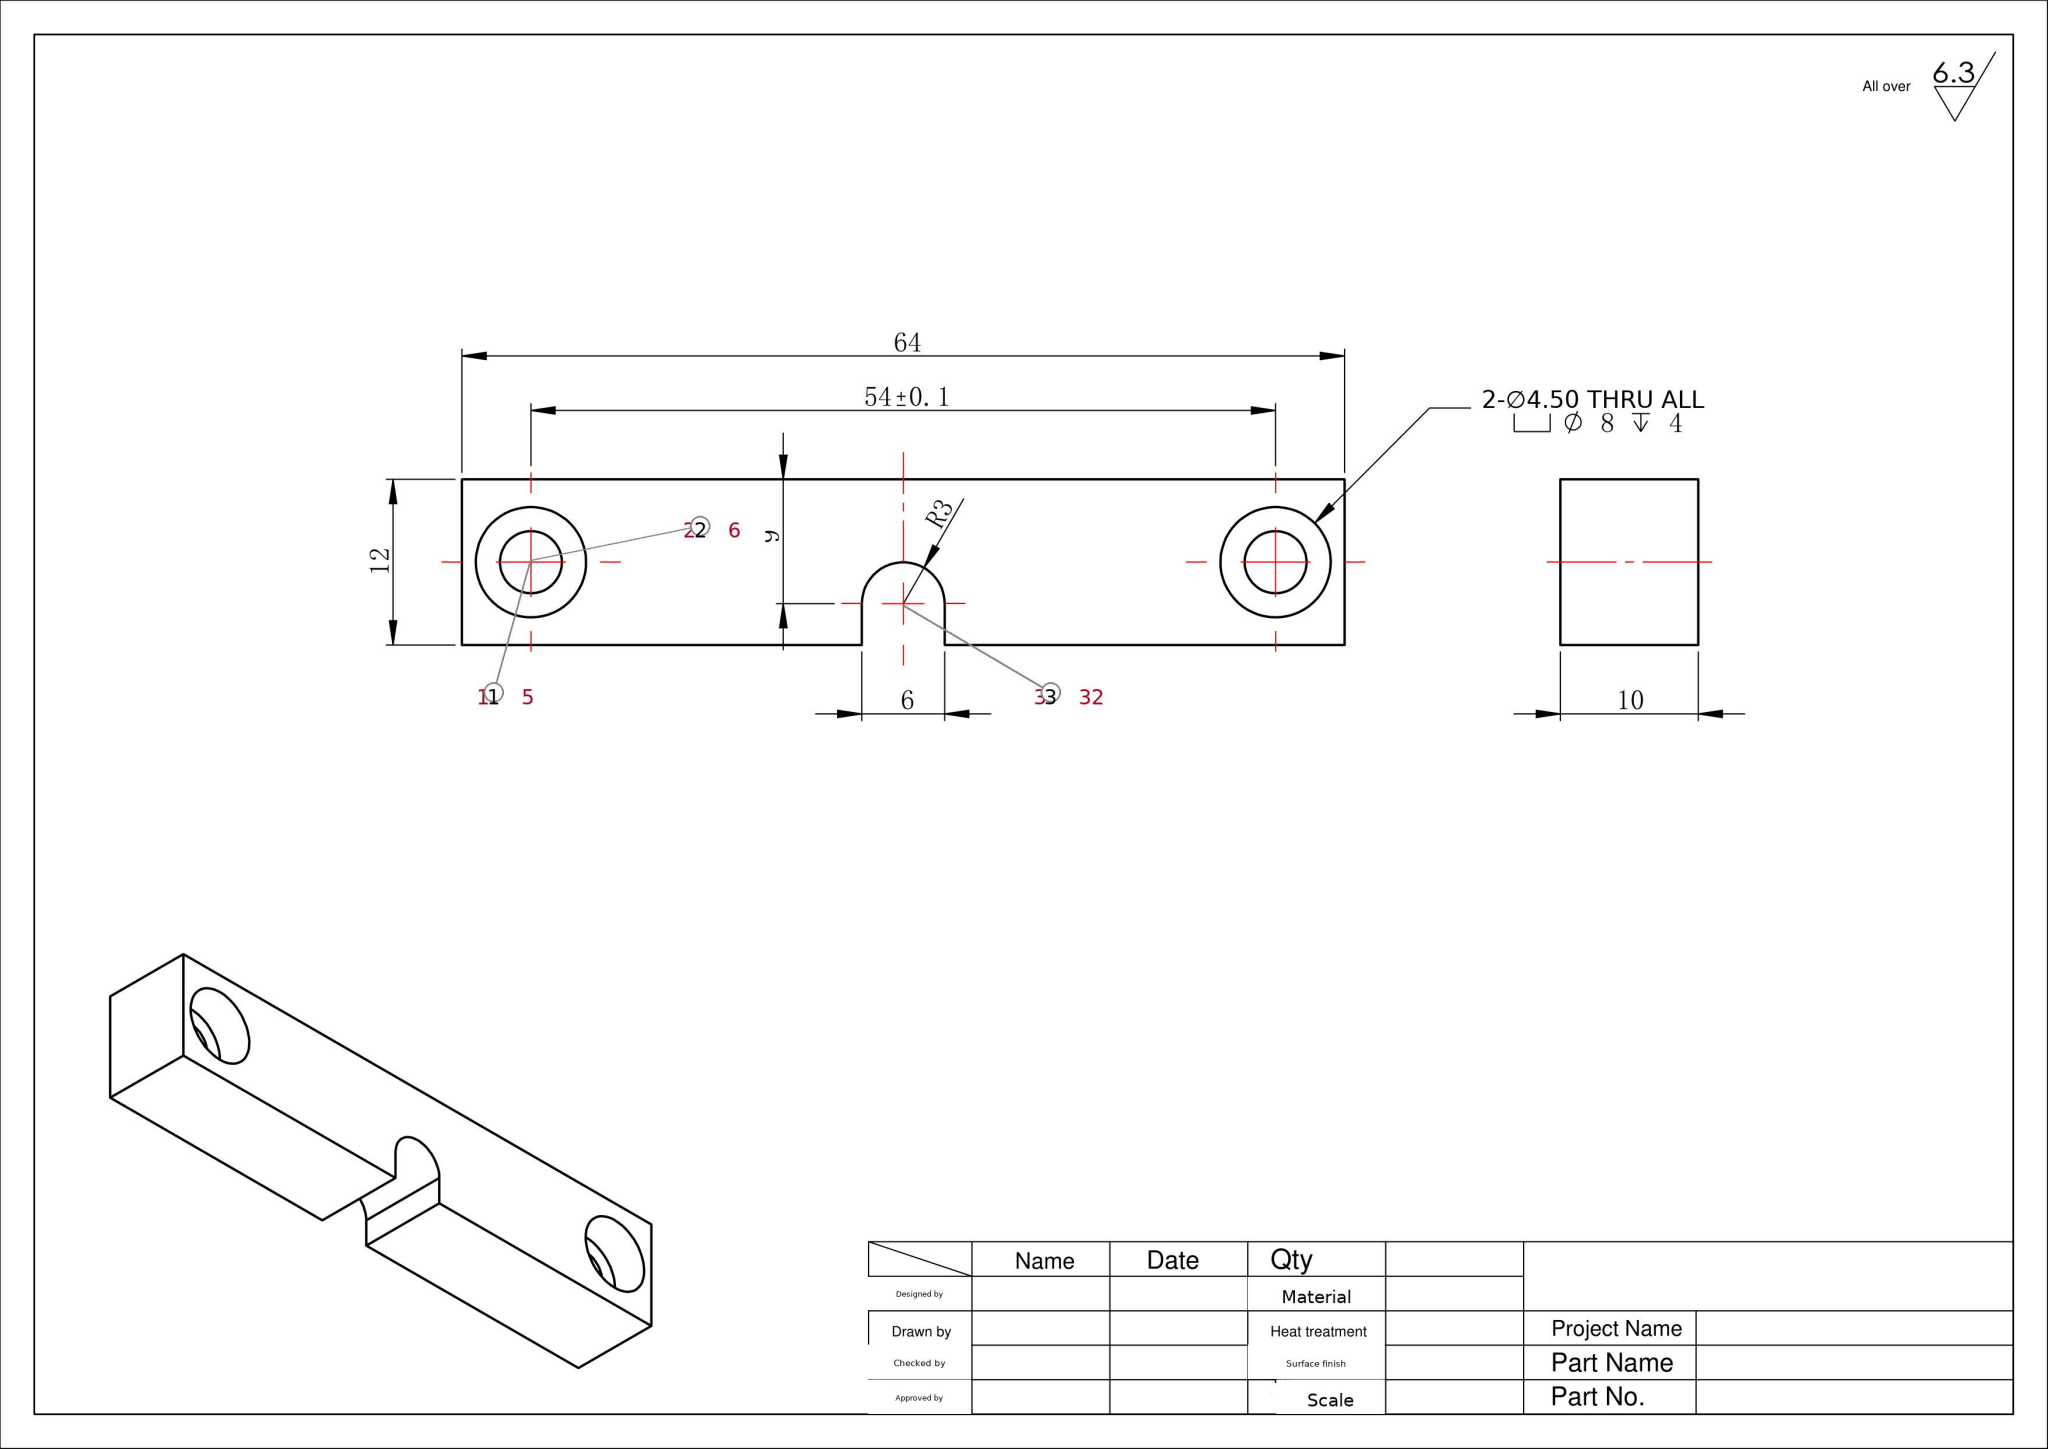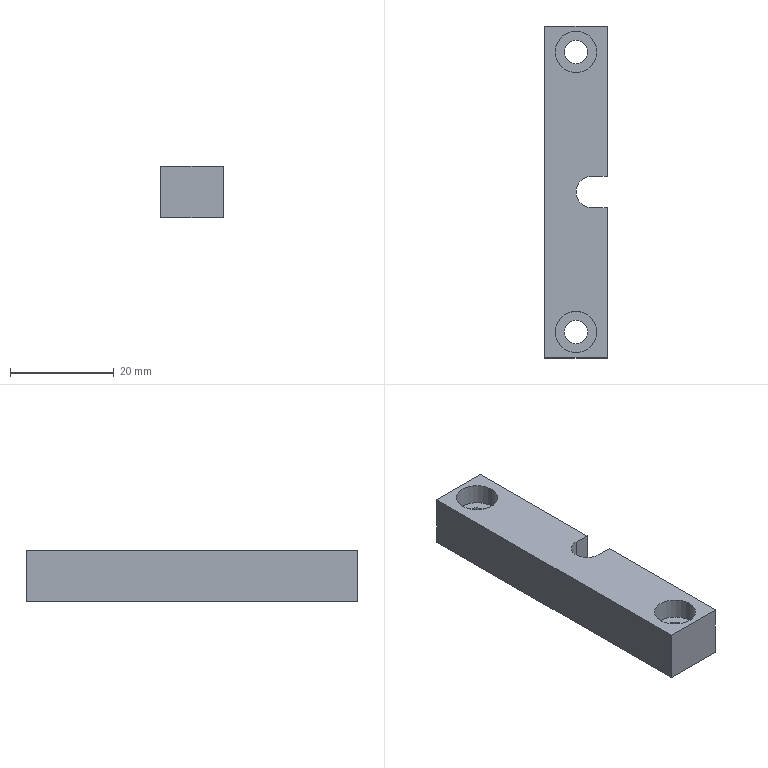Part | SolidWorks | mm | 1 solid | 20 faces | box 12 x 64 x 10 mm | volume 6766 mm3 | plane 11 | cylinder 9 | commonest cylinder face diameters 4.5 x4 8 x4 6 x1
build123d program:
from build123d import *

# Parameters (mm, degrees)
SKETCH1_W                                        = 12
SKETCH1_H                                        = 64
EXTRUDE1_DEPTH                                   = 10
CUT_EXTRUDE1_DEPTH                               = 66.879
M4_HEX_SOCKET_HEAD_CAP_SCREW_CBORE13_D           = 4.5
M4_HEX_SOCKET_HEAD_CAP_SCREW_CBORE13_CBORE_D     = 8
M4_HEX_SOCKET_HEAD_CAP_SCREW_CBORE13_CBORE_DEPTH = 4


with BuildPart() as part:
    # Sketch1 → Extrude1 (new body)
    with BuildSketch(Plane.XY):
        with Locations((6, 32)):
            Rectangle(SKETCH1_W, SKETCH1_H)
    extrude(amount=EXTRUDE1_DEPTH)

    # Sketch2 → Cut-Extrude1 (cut, through all)
    with BuildSketch(Plane.XY.offset(10)):
        with BuildLine():
            Line((9, 35), (14.637, 35))
            Line((14.637, 35), (14.637, 29))
            Line((14.637, 29), (9, 29))
            ThreePointArc((9, 29), (6, 32), (9, 35))
        make_face()
    extrude(amount=-CUT_EXTRUDE1_DEPTH, mode=Mode.SUBTRACT)

    # M4 Hex Socket Head Cap Screw CBORE13 (through all)
    with Locations(Plane(origin=(6, 59, 10), x_dir=(1, 0, 0), z_dir=(0, 0, 1))):
        with Locations((0, 0), (0, -54)):
            CounterBoreHole(M4_HEX_SOCKET_HEAD_CAP_SCREW_CBORE13_D / 2, M4_HEX_SOCKET_HEAD_CAP_SCREW_CBORE13_CBORE_D / 2, M4_HEX_SOCKET_HEAD_CAP_SCREW_CBORE13_CBORE_DEPTH)


solid = part.part
STEP:
#1=CARTESIAN_POINT('',(3.75,59.,0.));
#2=VERTEX_POINT('',#1);
#3=CARTESIAN_POINT('',(8.25,59.,0.));
#4=VERTEX_POINT('',#3);
#5=CARTESIAN_POINT('',(6.,59.,0.));
#6=DIRECTION('',(0.,0.,1.));
#7=DIRECTION('',(1.,0.,0.));
#8=AXIS2_PLACEMENT_3D('',#5,#6,#7);
#9=CIRCLE('',#8,2.25);
#10=EDGE_CURVE('',#2,#4,#9,.T.);
#11=ORIENTED_EDGE('',*,*,#10,.F.);
#12=CARTESIAN_POINT('',(3.75,59.,6.));
#13=VERTEX_POINT('',#12);
#14=CARTESIAN_POINT('',(3.75,59.,10.));
#15=DIRECTION('',(0.,0.,1.));
#16=VECTOR('',#15,1000.);
#17=LINE('',#14,#16);
#18=EDGE_CURVE('',#2,#13,#17,.T.);
#19=ORIENTED_EDGE('',*,*,#18,.T.);
#20=CARTESIAN_POINT('',(8.25,59.,6.));
#21=VERTEX_POINT('',#20);
#22=CARTESIAN_POINT('',(6.,59.,6.));
#23=DIRECTION('',(0.,0.,1.));
#24=DIRECTION('',(1.,0.,0.));
#25=AXIS2_PLACEMENT_3D('',#22,#23,#24);
#26=CIRCLE('',#25,2.25);
#27=EDGE_CURVE('',#13,#21,#26,.T.);
#28=ORIENTED_EDGE('',*,*,#27,.T.);
#29=CARTESIAN_POINT('',(8.25,59.,10.));
#30=DIRECTION('',(0.,0.,1.));
#31=VECTOR('',#30,1000.);
#32=LINE('',#29,#31);
#33=EDGE_CURVE('',#4,#21,#32,.T.);
#34=ORIENTED_EDGE('',*,*,#33,.F.);
#35=EDGE_LOOP('',(#11,#19,#28,#34));
#36=FACE_OUTER_BOUND('',#35,.T.);
#37=CARTESIAN_POINT('',(6.,59.,10.));
#38=DIRECTION('',(0.,0.,1.));
#39=DIRECTION('',(1.,0.,0.));
#40=AXIS2_PLACEMENT_3D('',#37,#38,#39);
#41=CYLINDRICAL_SURFACE('',#40,2.25);
#42=ADVANCED_FACE('',(#36),#41,.F.);
#43=CARTESIAN_POINT('',(2.,59.,6.));
#44=VERTEX_POINT('',#43);
#45=CARTESIAN_POINT('',(10.,59.,6.));
#46=VERTEX_POINT('',#45);
#47=CARTESIAN_POINT('',(6.,59.,6.));
#48=DIRECTION('',(0.,0.,1.));
#49=DIRECTION('',(1.,0.,0.));
#50=AXIS2_PLACEMENT_3D('',#47,#48,#49);
#51=CIRCLE('',#50,4.);
#52=EDGE_CURVE('',#44,#46,#51,.T.);
#53=ORIENTED_EDGE('',*,*,#52,.F.);
#54=CARTESIAN_POINT('',(2.,59.,10.));
#55=VERTEX_POINT('',#54);
#56=CARTESIAN_POINT('',(2.,59.,10.));
#57=DIRECTION('',(0.,0.,1.));
#58=VECTOR('',#57,1000.);
#59=LINE('',#56,#58);
#60=EDGE_CURVE('',#44,#55,#59,.T.);
#61=ORIENTED_EDGE('',*,*,#60,.T.);
#62=CARTESIAN_POINT('',(10.,59.,10.));
#63=VERTEX_POINT('',#62);
#64=CARTESIAN_POINT('',(6.,59.,10.));
#65=DIRECTION('',(0.,0.,1.));
#66=DIRECTION('',(1.,0.,0.));
#67=AXIS2_PLACEMENT_3D('',#64,#65,#66);
#68=CIRCLE('',#67,4.);
#69=EDGE_CURVE('',#55,#63,#68,.T.);
#70=ORIENTED_EDGE('',*,*,#69,.T.);
#71=CARTESIAN_POINT('',(10.,59.,10.));
#72=DIRECTION('',(0.,0.,1.));
#73=VECTOR('',#72,1000.);
#74=LINE('',#71,#73);
#75=EDGE_CURVE('',#46,#63,#74,.T.);
#76=ORIENTED_EDGE('',*,*,#75,.F.);
#77=EDGE_LOOP('',(#53,#61,#70,#76));
#78=FACE_OUTER_BOUND('',#77,.T.);
#79=CARTESIAN_POINT('',(6.,59.,10.));
#80=DIRECTION('',(0.,0.,1.));
#81=DIRECTION('',(1.,0.,0.));
#82=AXIS2_PLACEMENT_3D('',#79,#80,#81);
#83=CYLINDRICAL_SURFACE('',#82,4.);
#84=ADVANCED_FACE('',(#78),#83,.F.);
#85=CARTESIAN_POINT('',(3.75,5.,0.));
#86=VERTEX_POINT('',#85);
#87=CARTESIAN_POINT('',(8.25,5.,0.));
#88=VERTEX_POINT('',#87);
#89=CARTESIAN_POINT('',(6.,5.,0.));
#90=DIRECTION('',(0.,0.,1.));
#91=DIRECTION('',(1.,0.,0.));
#92=AXIS2_PLACEMENT_3D('',#89,#90,#91);
#93=CIRCLE('',#92,2.25);
#94=EDGE_CURVE('',#86,#88,#93,.T.);
#95=ORIENTED_EDGE('',*,*,#94,.F.);
#96=CARTESIAN_POINT('',(3.75,5.,6.));
#97=VERTEX_POINT('',#96);
#98=CARTESIAN_POINT('',(3.75,5.,10.));
#99=DIRECTION('',(0.,0.,1.));
#100=VECTOR('',#99,1000.);
#101=LINE('',#98,#100);
#102=EDGE_CURVE('',#86,#97,#101,.T.);
#103=ORIENTED_EDGE('',*,*,#102,.T.);
#104=CARTESIAN_POINT('',(8.25,5.,6.));
#105=VERTEX_POINT('',#104);
#106=CARTESIAN_POINT('',(6.,5.,6.));
#107=DIRECTION('',(0.,0.,1.));
#108=DIRECTION('',(1.,0.,0.));
#109=AXIS2_PLACEMENT_3D('',#106,#107,#108);
#110=CIRCLE('',#109,2.25);
#111=EDGE_CURVE('',#97,#105,#110,.T.);
#112=ORIENTED_EDGE('',*,*,#111,.T.);
#113=CARTESIAN_POINT('',(8.25,5.,10.));
#114=DIRECTION('',(0.,0.,1.));
#115=VECTOR('',#114,1000.);
#116=LINE('',#113,#115);
#117=EDGE_CURVE('',#88,#105,#116,.T.);
#118=ORIENTED_EDGE('',*,*,#117,.F.);
#119=EDGE_LOOP('',(#95,#103,#112,#118));
#120=FACE_OUTER_BOUND('',#119,.T.);
#121=CARTESIAN_POINT('',(6.,5.,10.));
#122=DIRECTION('',(0.,0.,1.));
#123=DIRECTION('',(1.,0.,0.));
#124=AXIS2_PLACEMENT_3D('',#121,#122,#123);
#125=CYLINDRICAL_SURFACE('',#124,2.25);
#126=ADVANCED_FACE('',(#120),#125,.F.);
#127=CARTESIAN_POINT('',(2.,5.,6.));
#128=VERTEX_POINT('',#127);
#129=CARTESIAN_POINT('',(10.,5.,6.));
#130=VERTEX_POINT('',#129);
#131=CARTESIAN_POINT('',(6.,5.,6.));
#132=DIRECTION('',(0.,0.,1.));
#133=DIRECTION('',(1.,0.,0.));
#134=AXIS2_PLACEMENT_3D('',#131,#132,#133);
#135=CIRCLE('',#134,4.);
#136=EDGE_CURVE('',#128,#130,#135,.T.);
#137=ORIENTED_EDGE('',*,*,#136,.F.);
#138=CARTESIAN_POINT('',(2.,5.,10.));
#139=VERTEX_POINT('',#138);
#140=CARTESIAN_POINT('',(2.,5.,10.));
#141=DIRECTION('',(0.,0.,1.));
#142=VECTOR('',#141,1000.);
#143=LINE('',#140,#142);
#144=EDGE_CURVE('',#128,#139,#143,.T.);
#145=ORIENTED_EDGE('',*,*,#144,.T.);
#146=CARTESIAN_POINT('',(10.,5.,10.));
#147=VERTEX_POINT('',#146);
#148=CARTESIAN_POINT('',(6.,5.,10.));
#149=DIRECTION('',(0.,0.,1.));
#150=DIRECTION('',(1.,0.,0.));
#151=AXIS2_PLACEMENT_3D('',#148,#149,#150);
#152=CIRCLE('',#151,4.);
#153=EDGE_CURVE('',#139,#147,#152,.T.);
#154=ORIENTED_EDGE('',*,*,#153,.T.);
#155=CARTESIAN_POINT('',(10.,5.,10.));
#156=DIRECTION('',(0.,0.,1.));
#157=VECTOR('',#156,1000.);
#158=LINE('',#155,#157);
#159=EDGE_CURVE('',#130,#147,#158,.T.);
#160=ORIENTED_EDGE('',*,*,#159,.F.);
#161=EDGE_LOOP('',(#137,#145,#154,#160));
#162=FACE_OUTER_BOUND('',#161,.T.);
#163=CARTESIAN_POINT('',(6.,5.,10.));
#164=DIRECTION('',(0.,0.,1.));
#165=DIRECTION('',(1.,0.,0.));
#166=AXIS2_PLACEMENT_3D('',#163,#164,#165);
#167=CYLINDRICAL_SURFACE('',#166,4.);
#168=ADVANCED_FACE('',(#162),#167,.F.);
#169=CARTESIAN_POINT('',(12.,35.,10.));
#170=VERTEX_POINT('',#169);
#171=CARTESIAN_POINT('',(12.,64.,10.));
#172=VERTEX_POINT('',#171);
#173=CARTESIAN_POINT('',(12.,0.,10.));
#174=DIRECTION('',(0.,1.,0.));
#175=VECTOR('',#174,1000.);
#176=LINE('',#173,#175);
#177=EDGE_CURVE('',#170,#172,#176,.T.);
#178=ORIENTED_EDGE('',*,*,#177,.F.);
#179=CARTESIAN_POINT('',(12.,35.,0.));
#180=VERTEX_POINT('',#179);
#181=CARTESIAN_POINT('',(12.,35.,10.));
#182=DIRECTION('',(0.,0.,-1.));
#183=VECTOR('',#182,1000.);
#184=LINE('',#181,#183);
#185=EDGE_CURVE('',#170,#180,#184,.T.);
#186=ORIENTED_EDGE('',*,*,#185,.T.);
#187=CARTESIAN_POINT('',(12.,64.,0.));
#188=VERTEX_POINT('',#187);
#189=CARTESIAN_POINT('',(12.,0.,0.));
#190=DIRECTION('',(0.,1.,0.));
#191=VECTOR('',#190,1000.);
#192=LINE('',#189,#191);
#193=EDGE_CURVE('',#180,#188,#192,.T.);
#194=ORIENTED_EDGE('',*,*,#193,.T.);
#195=CARTESIAN_POINT('',(12.,64.,10.));
#196=DIRECTION('',(0.,0.,-1.));
#197=VECTOR('',#196,1000.);
#198=LINE('',#195,#197);
#199=EDGE_CURVE('',#172,#188,#198,.T.);
#200=ORIENTED_EDGE('',*,*,#199,.F.);
#201=EDGE_LOOP('',(#178,#186,#194,#200));
#202=FACE_OUTER_BOUND('',#201,.T.);
#203=CARTESIAN_POINT('',(12.,0.,10.));
#204=DIRECTION('',(-1.,0.,0.));
#205=DIRECTION('',(0.,0.,1.));
#206=AXIS2_PLACEMENT_3D('',#203,#204,#205);
#207=PLANE('',#206);
#208=ADVANCED_FACE('',(#202),#207,.F.);
#209=CARTESIAN_POINT('',(0.,64.,0.));
#210=VERTEX_POINT('',#209);
#211=CARTESIAN_POINT('',(0.,0.,0.));
#212=VERTEX_POINT('',#211);
#213=CARTESIAN_POINT('',(0.,0.,0.));
#214=DIRECTION('',(0.,-1.,0.));
#215=VECTOR('',#214,1000.);
#216=LINE('',#213,#215);
#217=EDGE_CURVE('',#210,#212,#216,.T.);
#218=ORIENTED_EDGE('',*,*,#217,.T.);
#219=CARTESIAN_POINT('',(0.,0.,10.));
#220=VERTEX_POINT('',#219);
#221=CARTESIAN_POINT('',(0.,0.,10.));
#222=DIRECTION('',(0.,0.,-1.));
#223=VECTOR('',#222,1000.);
#224=LINE('',#221,#223);
#225=EDGE_CURVE('',#220,#212,#224,.T.);
#226=ORIENTED_EDGE('',*,*,#225,.F.);
#227=CARTESIAN_POINT('',(0.,64.,10.));
#228=VERTEX_POINT('',#227);
#229=CARTESIAN_POINT('',(0.,0.,10.));
#230=DIRECTION('',(0.,-1.,0.));
#231=VECTOR('',#230,1000.);
#232=LINE('',#229,#231);
#233=EDGE_CURVE('',#228,#220,#232,.T.);
#234=ORIENTED_EDGE('',*,*,#233,.F.);
#235=CARTESIAN_POINT('',(0.,64.,10.));
#236=DIRECTION('',(0.,0.,-1.));
#237=VECTOR('',#236,1000.);
#238=LINE('',#235,#237);
#239=EDGE_CURVE('',#228,#210,#238,.T.);
#240=ORIENTED_EDGE('',*,*,#239,.T.);
#241=EDGE_LOOP('',(#218,#226,#234,#240));
#242=FACE_OUTER_BOUND('',#241,.T.);
#243=CARTESIAN_POINT('',(0.,0.,10.));
#244=DIRECTION('',(1.,0.,0.));
#245=DIRECTION('',(0.,0.,-1.));
#246=AXIS2_PLACEMENT_3D('',#243,#244,#245);
#247=PLANE('',#246);
#248=ADVANCED_FACE('',(#242),#247,.F.);
#249=CARTESIAN_POINT('',(12.,0.,0.));
#250=VERTEX_POINT('',#249);
#251=CARTESIAN_POINT('',(0.,0.,0.));
#252=DIRECTION('',(1.,0.,0.));
#253=VECTOR('',#252,1000.);
#254=LINE('',#251,#253);
#255=EDGE_CURVE('',#212,#250,#254,.T.);
#256=ORIENTED_EDGE('',*,*,#255,.T.);
#257=CARTESIAN_POINT('',(12.,0.,10.));
#258=VERTEX_POINT('',#257);
#259=CARTESIAN_POINT('',(12.,0.,10.));
#260=DIRECTION('',(0.,0.,-1.));
#261=VECTOR('',#260,1000.);
#262=LINE('',#259,#261);
#263=EDGE_CURVE('',#258,#250,#262,.T.);
#264=ORIENTED_EDGE('',*,*,#263,.F.);
#265=CARTESIAN_POINT('',(0.,0.,10.));
#266=DIRECTION('',(1.,0.,0.));
#267=VECTOR('',#266,1000.);
#268=LINE('',#265,#267);
#269=EDGE_CURVE('',#220,#258,#268,.T.);
#270=ORIENTED_EDGE('',*,*,#269,.F.);
#271=ORIENTED_EDGE('',*,*,#225,.T.);
#272=EDGE_LOOP('',(#256,#264,#270,#271));
#273=FACE_OUTER_BOUND('',#272,.T.);
#274=CARTESIAN_POINT('',(0.,0.,10.));
#275=DIRECTION('',(0.,1.,0.));
#276=DIRECTION('',(0.,0.,1.));
#277=AXIS2_PLACEMENT_3D('',#274,#275,#276);
#278=PLANE('',#277);
#279=ADVANCED_FACE('',(#273),#278,.F.);
#280=CARTESIAN_POINT('',(12.,29.,0.));
#281=VERTEX_POINT('',#280);
#282=CARTESIAN_POINT('',(12.,0.,0.));
#283=DIRECTION('',(0.,1.,0.));
#284=VECTOR('',#283,1000.);
#285=LINE('',#282,#284);
#286=EDGE_CURVE('',#250,#281,#285,.T.);
#287=ORIENTED_EDGE('',*,*,#286,.T.);
#288=CARTESIAN_POINT('',(12.,29.,10.));
#289=VERTEX_POINT('',#288);
#290=CARTESIAN_POINT('',(12.,29.,10.));
#291=DIRECTION('',(0.,0.,1.));
#292=VECTOR('',#291,1000.);
#293=LINE('',#290,#292);
#294=EDGE_CURVE('',#281,#289,#293,.T.);
#295=ORIENTED_EDGE('',*,*,#294,.T.);
#296=CARTESIAN_POINT('',(12.,0.,10.));
#297=DIRECTION('',(0.,1.,0.));
#298=VECTOR('',#297,1000.);
#299=LINE('',#296,#298);
#300=EDGE_CURVE('',#258,#289,#299,.T.);
#301=ORIENTED_EDGE('',*,*,#300,.F.);
#302=ORIENTED_EDGE('',*,*,#263,.T.);
#303=EDGE_LOOP('',(#287,#295,#301,#302));
#304=FACE_OUTER_BOUND('',#303,.T.);
#305=CARTESIAN_POINT('',(12.,0.,10.));
#306=DIRECTION('',(-1.,0.,0.));
#307=DIRECTION('',(0.,0.,1.));
#308=AXIS2_PLACEMENT_3D('',#305,#306,#307);
#309=PLANE('',#308);
#310=ADVANCED_FACE('',(#304),#309,.F.);
#311=CARTESIAN_POINT('',(0.,64.,0.));
#312=DIRECTION('',(-1.,0.,0.));
#313=VECTOR('',#312,1000.);
#314=LINE('',#311,#313);
#315=EDGE_CURVE('',#188,#210,#314,.T.);
#316=ORIENTED_EDGE('',*,*,#315,.T.);
#317=ORIENTED_EDGE('',*,*,#239,.F.);
#318=CARTESIAN_POINT('',(0.,64.,10.));
#319=DIRECTION('',(-1.,0.,0.));
#320=VECTOR('',#319,1000.);
#321=LINE('',#318,#320);
#322=EDGE_CURVE('',#172,#228,#321,.T.);
#323=ORIENTED_EDGE('',*,*,#322,.F.);
#324=ORIENTED_EDGE('',*,*,#199,.T.);
#325=EDGE_LOOP('',(#316,#317,#323,#324));
#326=FACE_OUTER_BOUND('',#325,.T.);
#327=CARTESIAN_POINT('',(0.,64.,10.));
#328=DIRECTION('',(0.,-1.,0.));
#329=DIRECTION('',(0.,0.,-1.));
#330=AXIS2_PLACEMENT_3D('',#327,#328,#329);
#331=PLANE('',#330);
#332=ADVANCED_FACE('',(#326),#331,.F.);
#333=CARTESIAN_POINT('',(6.,59.,10.));
#334=DIRECTION('',(0.,0.,1.));
#335=DIRECTION('',(1.,0.,0.));
#336=AXIS2_PLACEMENT_3D('',#333,#334,#335);
#337=CIRCLE('',#336,4.);
#338=EDGE_CURVE('',#63,#55,#337,.T.);
#339=ORIENTED_EDGE('',*,*,#338,.F.);
#340=ORIENTED_EDGE('',*,*,#69,.F.);
#341=EDGE_LOOP('',(#339,#340));
#342=FACE_BOUND('',#341,.T.);
#343=CARTESIAN_POINT('',(6.,5.,10.));
#344=DIRECTION('',(0.,0.,1.));
#345=DIRECTION('',(1.,0.,0.));
#346=AXIS2_PLACEMENT_3D('',#343,#344,#345);
#347=CIRCLE('',#346,4.);
#348=EDGE_CURVE('',#147,#139,#347,.T.);
#349=ORIENTED_EDGE('',*,*,#348,.F.);
#350=ORIENTED_EDGE('',*,*,#153,.F.);
#351=EDGE_LOOP('',(#349,#350));
#352=FACE_BOUND('',#351,.T.);
#353=CARTESIAN_POINT('',(9.,35.,10.));
#354=VERTEX_POINT('',#353);
#355=CARTESIAN_POINT('',(9.,29.,10.));
#356=VERTEX_POINT('',#355);
#357=CARTESIAN_POINT('',(9.,32.,10.));
#358=DIRECTION('',(0.,0.,1.));
#359=DIRECTION('',(1.,0.,0.));
#360=AXIS2_PLACEMENT_3D('',#357,#358,#359);
#361=CIRCLE('',#360,3.);
#362=EDGE_CURVE('',#354,#356,#361,.T.);
#363=ORIENTED_EDGE('',*,*,#362,.F.);
#364=CARTESIAN_POINT('',(9.,35.,10.));
#365=DIRECTION('',(-1.,0.,0.));
#366=VECTOR('',#365,1000.);
#367=LINE('',#364,#366);
#368=EDGE_CURVE('',#170,#354,#367,.T.);
#369=ORIENTED_EDGE('',*,*,#368,.F.);
#370=ORIENTED_EDGE('',*,*,#177,.T.);
#371=ORIENTED_EDGE('',*,*,#322,.T.);
#372=ORIENTED_EDGE('',*,*,#233,.T.);
#373=ORIENTED_EDGE('',*,*,#269,.T.);
#374=ORIENTED_EDGE('',*,*,#300,.T.);
#375=CARTESIAN_POINT('',(14.637,29.,10.));
#376=DIRECTION('',(1.,0.,0.));
#377=VECTOR('',#376,1000.);
#378=LINE('',#375,#377);
#379=EDGE_CURVE('',#356,#289,#378,.T.);
#380=ORIENTED_EDGE('',*,*,#379,.F.);
#381=EDGE_LOOP('',(#363,#369,#370,#371,#372,#373,#374,#380));
#382=FACE_OUTER_BOUND('',#381,.T.);
#383=CARTESIAN_POINT('',(0.,64.,10.));
#384=DIRECTION('',(0.,0.,-1.));
#385=DIRECTION('',(-1.,0.,0.));
#386=AXIS2_PLACEMENT_3D('',#383,#384,#385);
#387=PLANE('',#386);
#388=ADVANCED_FACE('',(#342,#352,#382),#387,.F.);
#389=CARTESIAN_POINT('',(6.,59.,0.));
#390=DIRECTION('',(0.,0.,1.));
#391=DIRECTION('',(1.,0.,0.));
#392=AXIS2_PLACEMENT_3D('',#389,#390,#391);
#393=CIRCLE('',#392,2.25);
#394=EDGE_CURVE('',#4,#2,#393,.T.);
#395=ORIENTED_EDGE('',*,*,#394,.T.);
#396=ORIENTED_EDGE('',*,*,#10,.T.);
#397=EDGE_LOOP('',(#395,#396));
#398=FACE_BOUND('',#397,.T.);
#399=CARTESIAN_POINT('',(6.,5.,0.));
#400=DIRECTION('',(0.,0.,1.));
#401=DIRECTION('',(1.,0.,0.));
#402=AXIS2_PLACEMENT_3D('',#399,#400,#401);
#403=CIRCLE('',#402,2.25);
#404=EDGE_CURVE('',#88,#86,#403,.T.);
#405=ORIENTED_EDGE('',*,*,#404,.T.);
#406=ORIENTED_EDGE('',*,*,#94,.T.);
#407=EDGE_LOOP('',(#405,#406));
#408=FACE_BOUND('',#407,.T.);
#409=CARTESIAN_POINT('',(9.,35.,0.));
#410=VERTEX_POINT('',#409);
#411=CARTESIAN_POINT('',(0.,35.,0.));
#412=DIRECTION('',(1.,0.,0.));
#413=VECTOR('',#412,1000.);
#414=LINE('',#411,#413);
#415=EDGE_CURVE('',#410,#180,#414,.T.);
#416=ORIENTED_EDGE('',*,*,#415,.F.);
#417=CARTESIAN_POINT('',(9.,29.,0.));
#418=VERTEX_POINT('',#417);
#419=CARTESIAN_POINT('',(9.,32.,0.));
#420=DIRECTION('',(0.,0.,1.));
#421=DIRECTION('',(1.,0.,0.));
#422=AXIS2_PLACEMENT_3D('',#419,#420,#421);
#423=CIRCLE('',#422,3.);
#424=EDGE_CURVE('',#410,#418,#423,.T.);
#425=ORIENTED_EDGE('',*,*,#424,.T.);
#426=CARTESIAN_POINT('',(14.637,29.,0.));
#427=DIRECTION('',(1.,0.,0.));
#428=VECTOR('',#427,1000.);
#429=LINE('',#426,#428);
#430=EDGE_CURVE('',#418,#281,#429,.T.);
#431=ORIENTED_EDGE('',*,*,#430,.T.);
#432=ORIENTED_EDGE('',*,*,#286,.F.);
#433=ORIENTED_EDGE('',*,*,#255,.F.);
#434=ORIENTED_EDGE('',*,*,#217,.F.);
#435=ORIENTED_EDGE('',*,*,#315,.F.);
#436=ORIENTED_EDGE('',*,*,#193,.F.);
#437=EDGE_LOOP('',(#416,#425,#431,#432,#433,#434,#435,#436));
#438=FACE_OUTER_BOUND('',#437,.T.);
#439=CARTESIAN_POINT('',(0.,64.,0.));
#440=DIRECTION('',(0.,0.,-1.));
#441=DIRECTION('',(-1.,0.,0.));
#442=AXIS2_PLACEMENT_3D('',#439,#440,#441);
#443=PLANE('',#442);
#444=ADVANCED_FACE('',(#398,#408,#438),#443,.T.);
#445=ORIENTED_EDGE('',*,*,#368,.T.);
#446=CARTESIAN_POINT('',(9.,35.,0.));
#447=DIRECTION('',(0.,0.,1.));
#448=VECTOR('',#447,1000.);
#449=LINE('',#446,#448);
#450=EDGE_CURVE('',#410,#354,#449,.T.);
#451=ORIENTED_EDGE('',*,*,#450,.F.);
#452=ORIENTED_EDGE('',*,*,#415,.T.);
#453=ORIENTED_EDGE('',*,*,#185,.F.);
#454=EDGE_LOOP('',(#445,#451,#452,#453));
#455=FACE_OUTER_BOUND('',#454,.T.);
#456=CARTESIAN_POINT('',(9.,35.,0.));
#457=DIRECTION('',(0.,1.,0.));
#458=DIRECTION('',(0.,0.,1.));
#459=AXIS2_PLACEMENT_3D('',#456,#457,#458);
#460=PLANE('',#459);
#461=ADVANCED_FACE('',(#455),#460,.F.);
#462=ORIENTED_EDGE('',*,*,#430,.F.);
#463=CARTESIAN_POINT('',(9.,29.,0.));
#464=DIRECTION('',(0.,0.,1.));
#465=VECTOR('',#464,1000.);
#466=LINE('',#463,#465);
#467=EDGE_CURVE('',#418,#356,#466,.T.);
#468=ORIENTED_EDGE('',*,*,#467,.T.);
#469=ORIENTED_EDGE('',*,*,#379,.T.);
#470=ORIENTED_EDGE('',*,*,#294,.F.);
#471=EDGE_LOOP('',(#462,#468,#469,#470));
#472=FACE_OUTER_BOUND('',#471,.T.);
#473=CARTESIAN_POINT('',(14.637,29.,0.));
#474=DIRECTION('',(0.,-1.,0.));
#475=DIRECTION('',(1.,0.,0.));
#476=AXIS2_PLACEMENT_3D('',#473,#474,#475);
#477=PLANE('',#476);
#478=ADVANCED_FACE('',(#472),#477,.F.);
#479=ORIENTED_EDGE('',*,*,#362,.T.);
#480=ORIENTED_EDGE('',*,*,#467,.F.);
#481=ORIENTED_EDGE('',*,*,#424,.F.);
#482=ORIENTED_EDGE('',*,*,#450,.T.);
#483=EDGE_LOOP('',(#479,#480,#481,#482));
#484=FACE_OUTER_BOUND('',#483,.T.);
#485=CARTESIAN_POINT('',(9.,32.,0.));
#486=DIRECTION('',(0.,0.,1.));
#487=DIRECTION('',(1.,0.,0.));
#488=AXIS2_PLACEMENT_3D('',#485,#486,#487);
#489=CYLINDRICAL_SURFACE('',#488,3.);
#490=ADVANCED_FACE('',(#484),#489,.F.);
#491=ORIENTED_EDGE('',*,*,#144,.F.);
#492=CARTESIAN_POINT('',(6.,5.,6.));
#493=DIRECTION('',(0.,0.,1.));
#494=DIRECTION('',(1.,0.,0.));
#495=AXIS2_PLACEMENT_3D('',#492,#493,#494);
#496=CIRCLE('',#495,4.);
#497=EDGE_CURVE('',#130,#128,#496,.T.);
#498=ORIENTED_EDGE('',*,*,#497,.F.);
#499=ORIENTED_EDGE('',*,*,#159,.T.);
#500=ORIENTED_EDGE('',*,*,#348,.T.);
#501=EDGE_LOOP('',(#491,#498,#499,#500));
#502=FACE_OUTER_BOUND('',#501,.T.);
#503=CARTESIAN_POINT('',(6.,5.,10.));
#504=DIRECTION('',(0.,0.,1.));
#505=DIRECTION('',(1.,0.,0.));
#506=AXIS2_PLACEMENT_3D('',#503,#504,#505);
#507=CYLINDRICAL_SURFACE('',#506,4.);
#508=ADVANCED_FACE('',(#502),#507,.F.);
#509=CARTESIAN_POINT('',(6.,5.,6.));
#510=DIRECTION('',(0.,0.,1.));
#511=DIRECTION('',(1.,0.,0.));
#512=AXIS2_PLACEMENT_3D('',#509,#510,#511);
#513=CIRCLE('',#512,2.25);
#514=EDGE_CURVE('',#105,#97,#513,.T.);
#515=ORIENTED_EDGE('',*,*,#514,.F.);
#516=ORIENTED_EDGE('',*,*,#111,.F.);
#517=EDGE_LOOP('',(#515,#516));
#518=FACE_BOUND('',#517,.T.);
#519=ORIENTED_EDGE('',*,*,#497,.T.);
#520=ORIENTED_EDGE('',*,*,#136,.T.);
#521=EDGE_LOOP('',(#519,#520));
#522=FACE_OUTER_BOUND('',#521,.T.);
#523=CARTESIAN_POINT('',(8.25,5.,6.));
#524=DIRECTION('',(0.,0.,-1.));
#525=DIRECTION('',(-1.,0.,0.));
#526=AXIS2_PLACEMENT_3D('',#523,#524,#525);
#527=PLANE('',#526);
#528=ADVANCED_FACE('',(#518,#522),#527,.F.);
#529=ORIENTED_EDGE('',*,*,#102,.F.);
#530=ORIENTED_EDGE('',*,*,#404,.F.);
#531=ORIENTED_EDGE('',*,*,#117,.T.);
#532=ORIENTED_EDGE('',*,*,#514,.T.);
#533=EDGE_LOOP('',(#529,#530,#531,#532));
#534=FACE_OUTER_BOUND('',#533,.T.);
#535=CARTESIAN_POINT('',(6.,5.,10.));
#536=DIRECTION('',(0.,0.,1.));
#537=DIRECTION('',(1.,0.,0.));
#538=AXIS2_PLACEMENT_3D('',#535,#536,#537);
#539=CYLINDRICAL_SURFACE('',#538,2.25);
#540=ADVANCED_FACE('',(#534),#539,.F.);
#541=ORIENTED_EDGE('',*,*,#60,.F.);
#542=CARTESIAN_POINT('',(6.,59.,6.));
#543=DIRECTION('',(0.,0.,1.));
#544=DIRECTION('',(1.,0.,0.));
#545=AXIS2_PLACEMENT_3D('',#542,#543,#544);
#546=CIRCLE('',#545,4.);
#547=EDGE_CURVE('',#46,#44,#546,.T.);
#548=ORIENTED_EDGE('',*,*,#547,.F.);
#549=ORIENTED_EDGE('',*,*,#75,.T.);
#550=ORIENTED_EDGE('',*,*,#338,.T.);
#551=EDGE_LOOP('',(#541,#548,#549,#550));
#552=FACE_OUTER_BOUND('',#551,.T.);
#553=CARTESIAN_POINT('',(6.,59.,10.));
#554=DIRECTION('',(0.,0.,1.));
#555=DIRECTION('',(1.,0.,0.));
#556=AXIS2_PLACEMENT_3D('',#553,#554,#555);
#557=CYLINDRICAL_SURFACE('',#556,4.);
#558=ADVANCED_FACE('',(#552),#557,.F.);
#559=CARTESIAN_POINT('',(6.,59.,6.));
#560=DIRECTION('',(0.,0.,1.));
#561=DIRECTION('',(1.,0.,0.));
#562=AXIS2_PLACEMENT_3D('',#559,#560,#561);
#563=CIRCLE('',#562,2.25);
#564=EDGE_CURVE('',#21,#13,#563,.T.);
#565=ORIENTED_EDGE('',*,*,#564,.F.);
#566=ORIENTED_EDGE('',*,*,#27,.F.);
#567=EDGE_LOOP('',(#565,#566));
#568=FACE_BOUND('',#567,.T.);
#569=ORIENTED_EDGE('',*,*,#547,.T.);
#570=ORIENTED_EDGE('',*,*,#52,.T.);
#571=EDGE_LOOP('',(#569,#570));
#572=FACE_OUTER_BOUND('',#571,.T.);
#573=CARTESIAN_POINT('',(8.25,59.,6.));
#574=DIRECTION('',(0.,0.,-1.));
#575=DIRECTION('',(-1.,0.,0.));
#576=AXIS2_PLACEMENT_3D('',#573,#574,#575);
#577=PLANE('',#576);
#578=ADVANCED_FACE('',(#568,#572),#577,.F.);
#579=ORIENTED_EDGE('',*,*,#18,.F.);
#580=ORIENTED_EDGE('',*,*,#394,.F.);
#581=ORIENTED_EDGE('',*,*,#33,.T.);
#582=ORIENTED_EDGE('',*,*,#564,.T.);
#583=EDGE_LOOP('',(#579,#580,#581,#582));
#584=FACE_OUTER_BOUND('',#583,.T.);
#585=CARTESIAN_POINT('',(6.,59.,10.));
#586=DIRECTION('',(0.,0.,1.));
#587=DIRECTION('',(1.,0.,0.));
#588=AXIS2_PLACEMENT_3D('',#585,#586,#587);
#589=CYLINDRICAL_SURFACE('',#588,2.25);
#590=ADVANCED_FACE('',(#584),#589,.F.);
#591=CLOSED_SHELL('',(#42,#84,#126,#168,#208,#248,#279,#310,#332,#388,#444,#461,#478,#490,#508,#528,#540,#558,#578,#590));
#592=MANIFOLD_SOLID_BREP('',#591);
#593=CARTESIAN_POINT('',(0.,0.,0.));
#594=DIRECTION('',(0.,0.,1.));
#595=DIRECTION('',(1.,0.,0.));
#596=AXIS2_PLACEMENT_3D('',#593,#594,#595);
#597=(LENGTH_UNIT()NAMED_UNIT(*)SI_UNIT(.MILLI.,.METRE.));
#598=UNCERTAINTY_MEASURE_WITH_UNIT(LENGTH_MEASURE(0.00001),#597,'','');
#599=(NAMED_UNIT(*)PLANE_ANGLE_UNIT()SI_UNIT($,.RADIAN.));
#600=(NAMED_UNIT(*)SI_UNIT($,.STERADIAN.)SOLID_ANGLE_UNIT());
#601=(GEOMETRIC_REPRESENTATION_CONTEXT(3)GLOBAL_UNCERTAINTY_ASSIGNED_CONTEXT((#598))GLOBAL_UNIT_ASSIGNED_CONTEXT((#597,#599,#600))REPRESENTATION_CONTEXT('',''));
#602=ADVANCED_BREP_SHAPE_REPRESENTATION('',(#592,#596),#601);